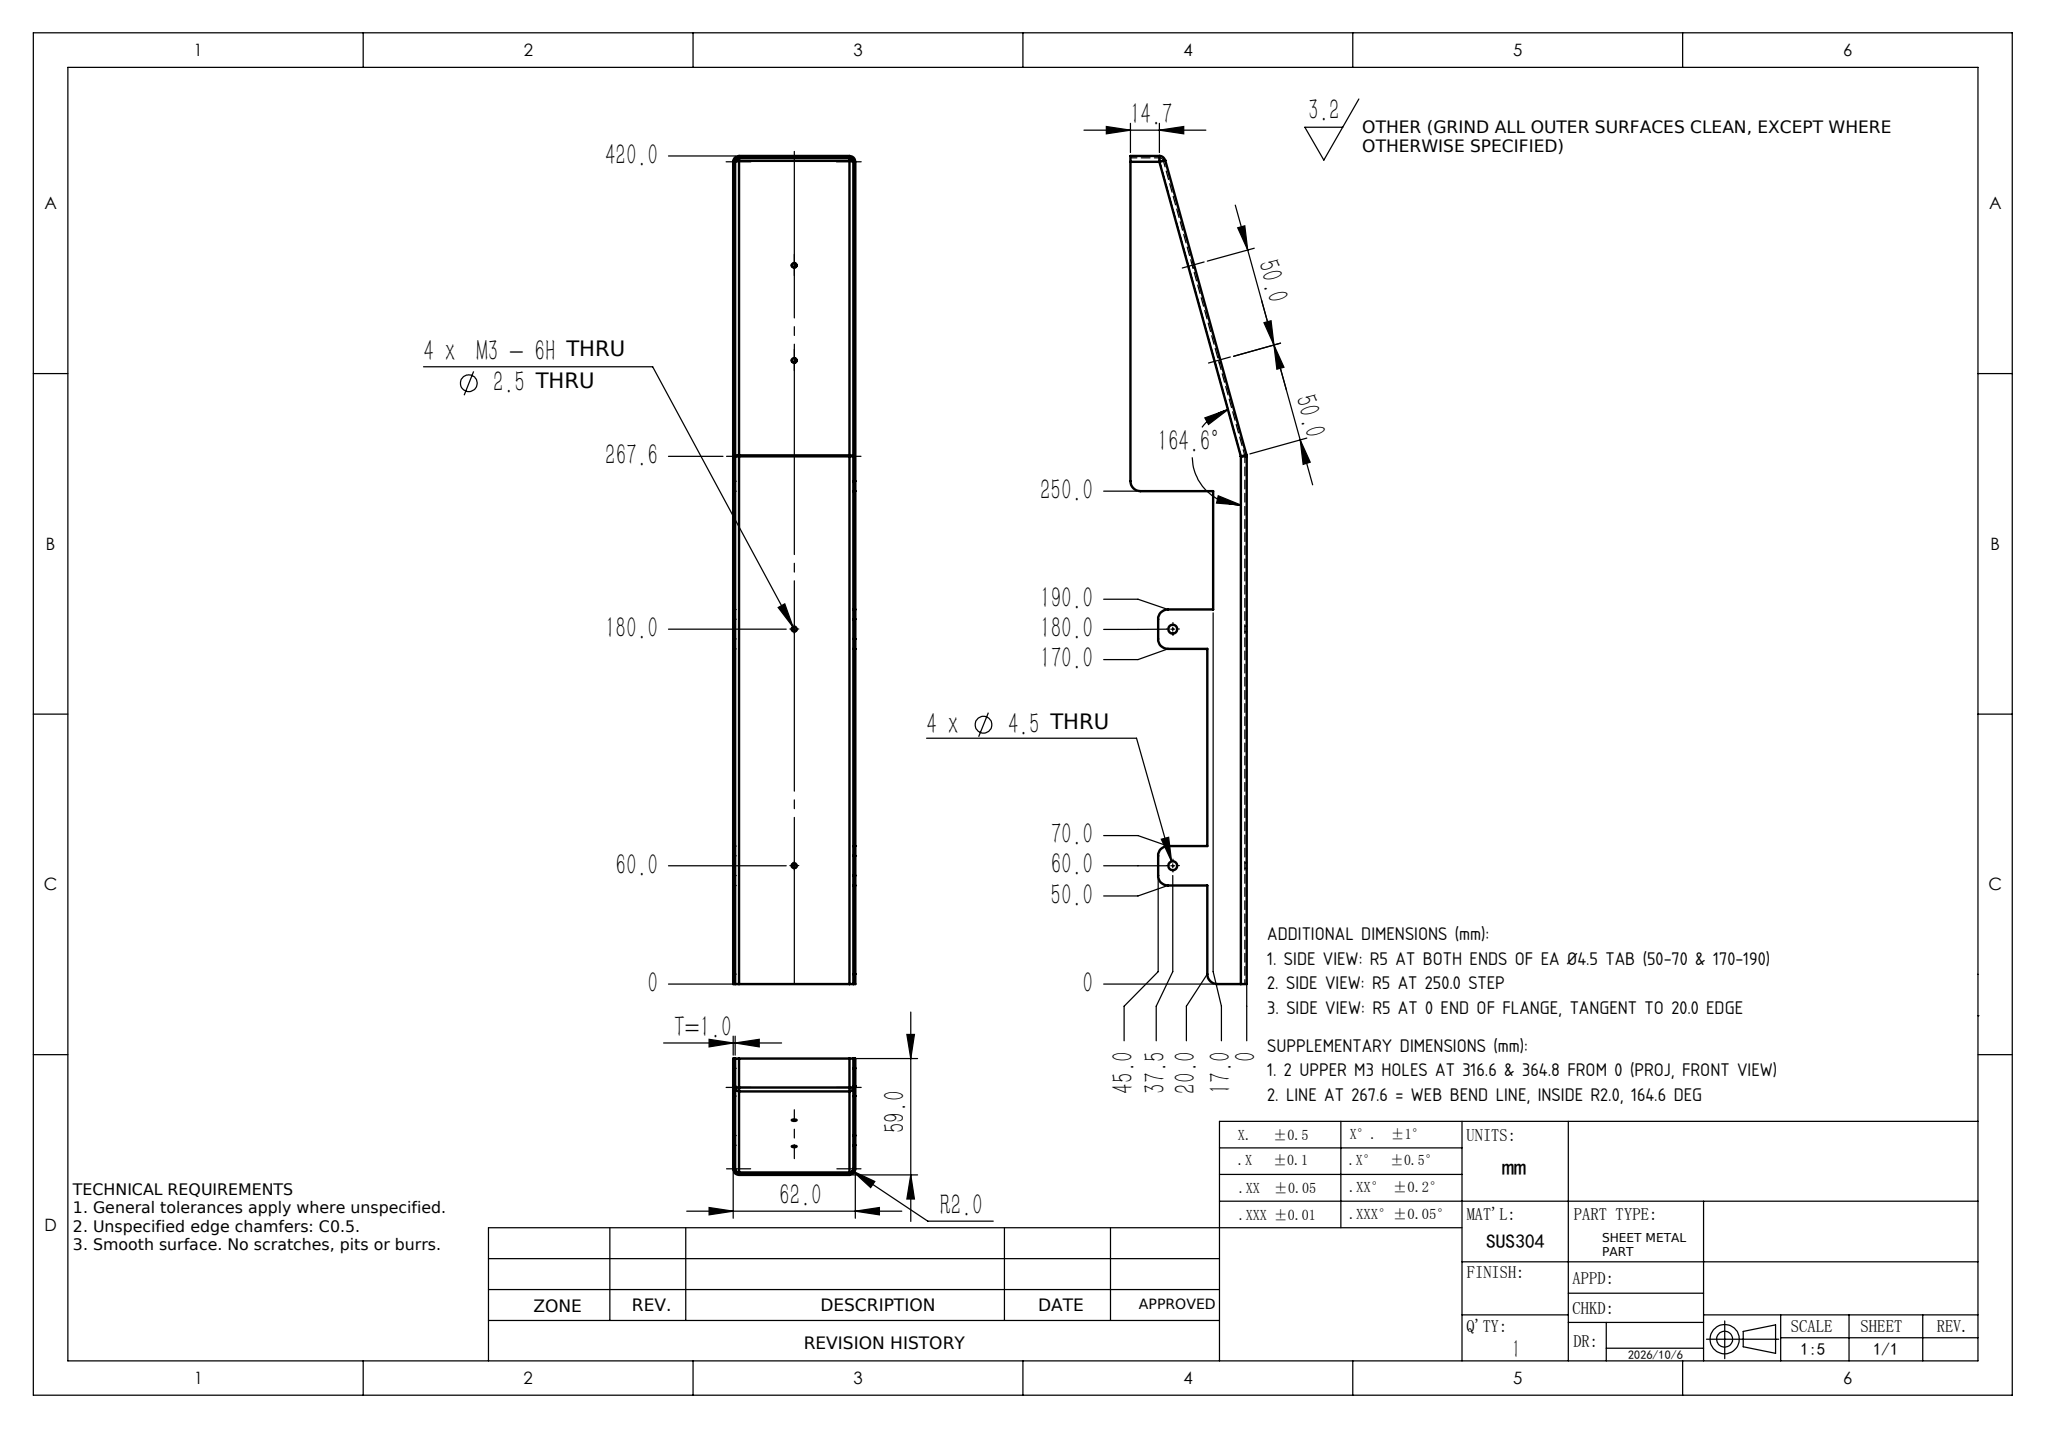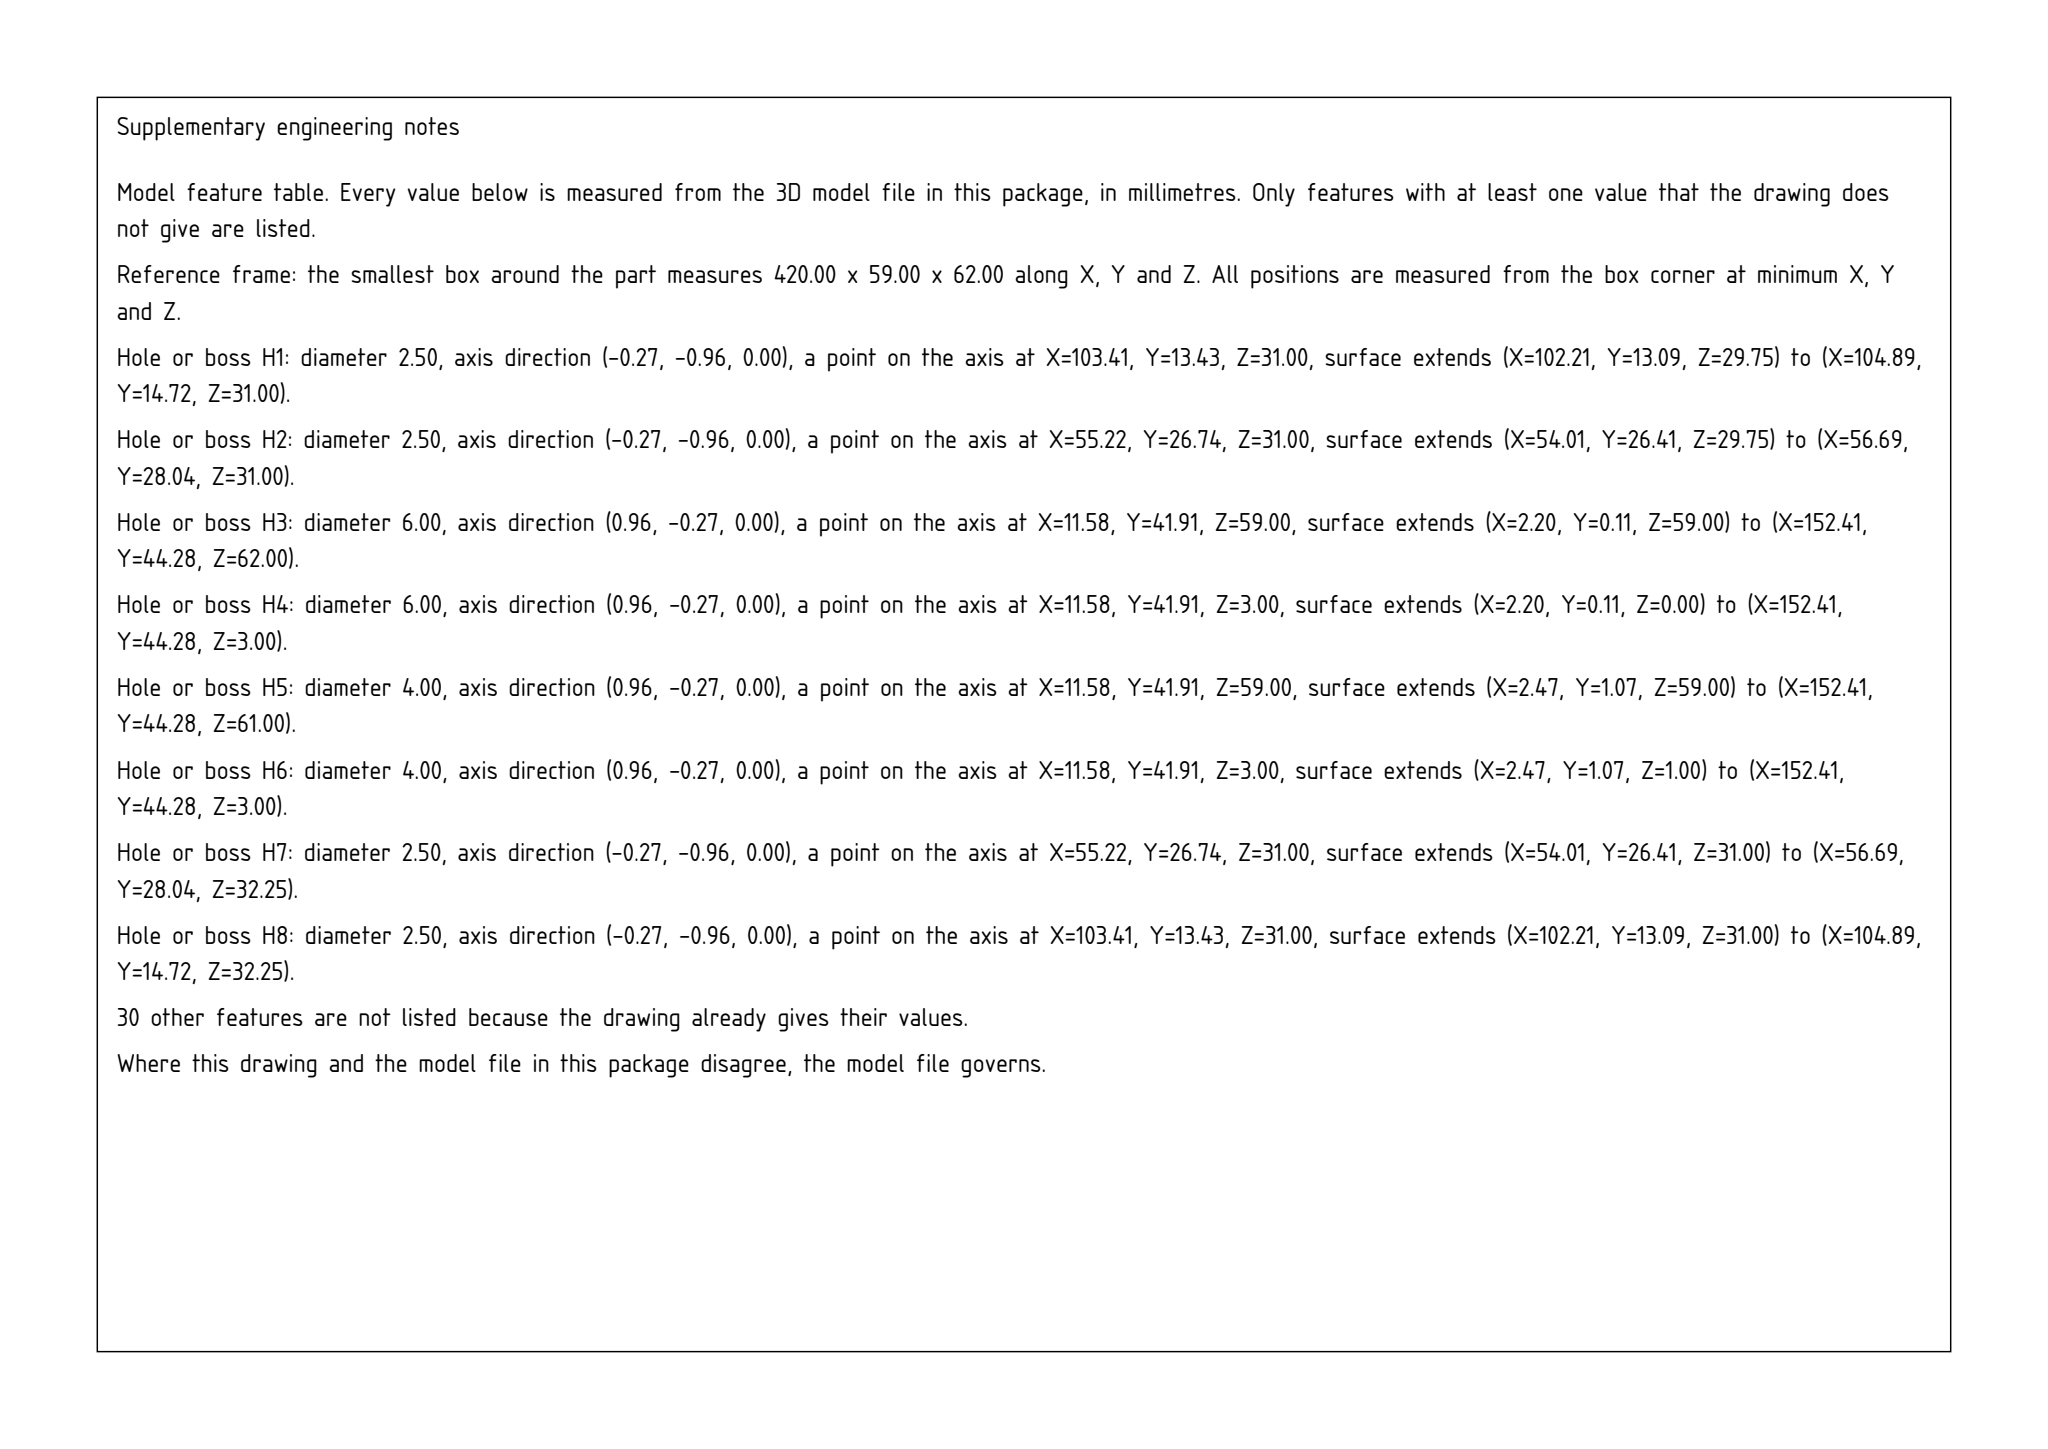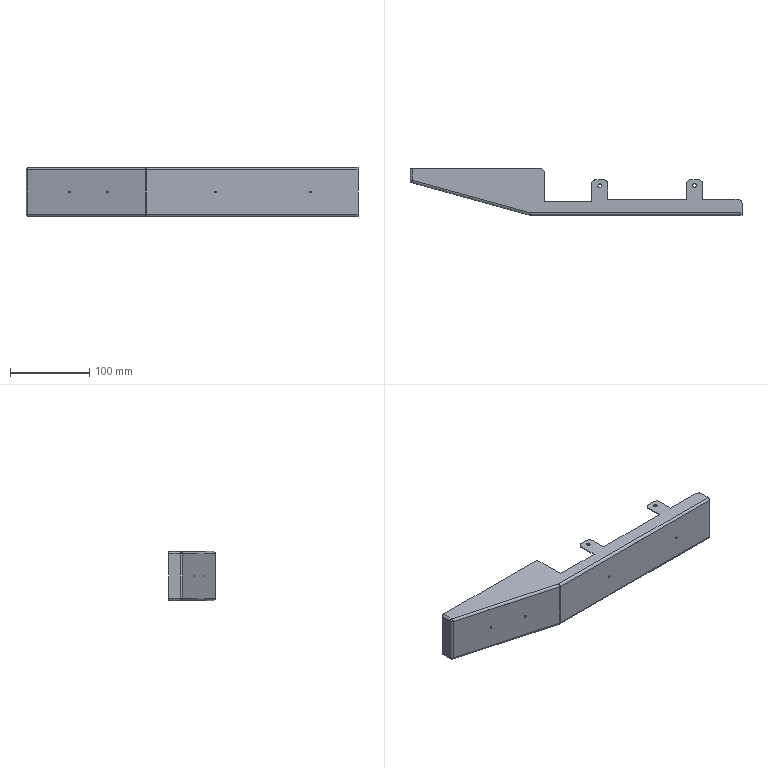Part | SolidWorks | mm | 1 solid | 84 faces | box 420 x 59 x 62 mm | volume 50692 mm3 | cylinder 44 | plane 32 | sphere 8 | commonest cylinder face diameters 10 x12 2.5 x8 4.5 x8 6 x8 4 x8
build123d program:
from build123d import *

# Parameters (mm, degrees)
SKETCH1_W            = 420
SKETCH1_H            = 59
BOSS_EXTRUDE1_DEPTH  = 31
CHAMFER1_SIZE        = 42
CHAMFER1_SIZE2       = 152
FILLET1_R            = 3
SHELL1_T             = -1
SKETCH2_W            = 50
SKETCH2_H            = 39
SKETCH2_W_2          = 100
SKETCH2_W_3          = 60
CUT_EXTRUDE1_DEPTH   = 429.632
SKETCH4_W            = 140
SKETCH4_H            = 14
CUT_EXTRUDE2_DEPTH   = 429.632
CUT_EXTRUDE3_DEPTH   = 425.268
M4_CLEARANCE_HOLE1_D = 4.5
SKETCH8_W            = 60
SKETCH8_H            = 3
CUT_EXTRUDE4_DEPTH   = 107
M3_TAPPED_HOLE1_D    = 2.5
M3_TAPPED_HOLE2_D    = 2.5
FILLET2_R            = 5


with BuildPart() as part:
    # Sketch1 → Boss-Extrude1 (new, symmetric)
    with BuildSketch(Plane.XY):
        with Locations((210, 29.5)):
            Rectangle(SKETCH1_W, SKETCH1_H)
    extrude(amount=BOSS_EXTRUDE1_DEPTH, both=True)

    # Chamfer1
    chamfer1_edges = [part.edges().sort_by_distance(p)[0] for p in [
        (0, 0, 0),
    ]]
    chamfer1_side = [part.faces().sort_by_distance(p)[0] for p in [
        (0, 29.5, 0),
    ]]
    chamfer(chamfer1_edges, length=CHAMFER1_SIZE, length2=CHAMFER1_SIZE2, reference=chamfer1_side[0])

    # Fillet1
    fillet1_edges = [part.edges().sort_by_distance(p)[0] for p in [
        (286, 0, -31),
        (286, 0, 31),
        (152, 0, 0),
        (76, 21, -31),
        (0, 42, 0),
        (76, 21, 31),
        (0, 50.5, 31),
        (0, 50.5, -31),
    ]]
    fillet(fillet1_edges, radius=FILLET1_R)

    # Shell1
    shell1_openings = [part.faces().sort_by_distance(p)[0] for p in [
        (210.031, 59, 0),
    ]]
    offset(amount=SHELL1_T, openings=shell1_openings, kind=Kind.INTERSECTION)

    # Sketch2 → Cut-Extrude1 (cut, through all)
    with BuildSketch(Plane.XY.offset(31)):
        with Locations((395, 39.5)):
            Rectangle(SKETCH2_W, SKETCH2_H)
        with Locations((300, 39.5)):
            Rectangle(SKETCH2_W_2, SKETCH2_H)
        with Locations((200, 39.5)):
            Rectangle(SKETCH2_W_3, SKETCH2_H)
    extrude(amount=-CUT_EXTRUDE1_DEPTH, mode=Mode.SUBTRACT)

    # Sketch4 → Cut-Extrude2 (cut, through all)
    with BuildSketch(Plane.XY.offset(31)):
        with Locations((300, 52)):
            Rectangle(SKETCH4_W, SKETCH4_H)
    extrude(amount=-CUT_EXTRUDE2_DEPTH, mode=Mode.SUBTRACT)

    # Sketch5 → Cut-Extrude3 (cut, through all)
    with BuildSketch(Plane.ZY.offset(-419)):
        with BuildLine():
            Line((30, 20), (-30, 20))
            Line((-30, 20), (-30, 3))
            ThreePointArc((-30, 3), (-29.414, 1.586), (-28, 1))
            Line((-28, 1), (28, 1))
            ThreePointArc((28, 1), (29.414, 1.586), (30, 3))
            Line((30, 3), (30, 20))
        make_face()
    extrude(amount=-CUT_EXTRUDE3_DEPTH, mode=Mode.SUBTRACT)

    # M4 Clearance Hole1 (through all)
    with Locations(Plane.XY.offset(31)):
        with Locations((240, 37.5), (360, 37.5)):
            Hole(M4_CLEARANCE_HOLE1_D / 2)

    # Sketch8 → Cut-Extrude4 (cut)
    with BuildSketch(Plane.XY.offset(31)):
        with Locations((200, 18.5)):
            Rectangle(SKETCH8_W, SKETCH8_H)
    extrude(amount=-CUT_EXTRUDE4_DEPTH, mode=Mode.SUBTRACT)

    # M3 Tapped Hole1 (through all)
    with Locations(Plane(origin=(10.782, 39.021, 0), x_dir=(-0.9639, 0.2663, 0), z_dir=(-0.2663, -0.9639, 0))):
        with Locations((-96.103, 0), (-46.103, 0)):
            Hole(M3_TAPPED_HOLE1_D / 2)

    # M3 Tapped Hole2 (through all)
    with Locations(Plane(origin=(240, 0, 0), x_dir=(0, 0, -1), z_dir=(0, -1, 0))):
        with Locations((0, 0), (0, 120)):
            Hole(M3_TAPPED_HOLE2_D / 2)

    # Fillet2
    fillet2_edges = [part.edges().sort_by_distance(p)[0] for p in [
        (170, 59, -30.5),
        (170, 59, 30.5),
        (250, 45, 30.5),
        (230, 45, -30.5),
        (250, 45, -30.5),
        (370, 45, -30.5),
        (350, 45, -30.5),
        (370, 45, 30.5),
        (350, 45, 30.5),
        (230, 45, 30.5),
        (420, 20, 30.5),
        (420, 20, -30.5),
    ]]
    fillet(fillet2_edges, radius=FILLET2_R)


solid = part.part